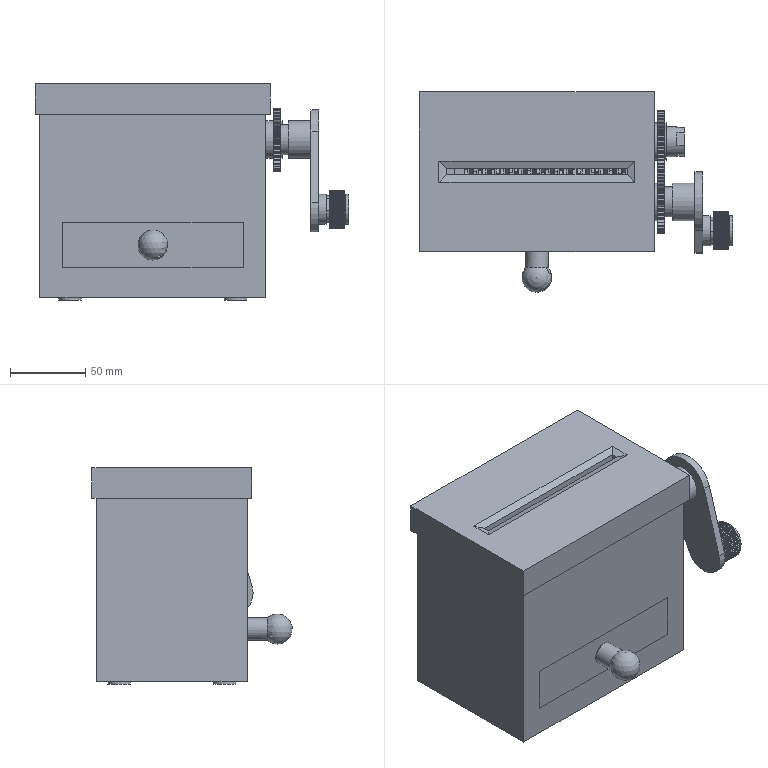Assembly | NX | mm | 9 component files | 11 solids | 2096 faces | box 208 x 133 x 143.5 mm | volume 1028833 mm3 | plane 897 | cylinder 878 | other 320 | sphere 1 | commonest cylinder face diameters 50 x288 1 x288 37.5 x80 42 x80 20 x56 25 x54 18 x8 15 x6
Bill of materials:
unnamed part 1 | 2 |  | Cylindrical shaft with a row of about 18 thin, evenly spaced discs along most of its length. Each disc has notched/serrated edges. Plain shaft stubs extend from both ends; one stub is longer and stepped, with a circumferential line or groove near its end.
unnamed part 2 | 1 |  | Flat, tapered lever arm with rounded ends. A plain cylindrical boss sits on one face at the wider end. A stepped cylindrical boss sits on the opposite face at the narrower end; it has a fine knurled or splined band and a smaller plain end cap.
unnamed part 3 | 1 |  | Open-top rectangular tray with thin walls and a flat floor. A short cylindrical stub ending in a sphere sticks out horizontally from the middle of one long outer wall. Small notches or tabs appear on the top edge of that wall, above the stub.
unnamed part 4 | 1 |  | Flat rectangular plate with one long, narrow through-slot running parallel to its long edge. The slot edges are chamfered or tapered on the top face.
unnamed part 5 | 2 |  | Spur gear with about 40 straight teeth around a large central bore. The bore has a small rectangular keyway notch. A cylindrical hub projects from one face.
unnamed part 6 | 1 |  | Thin, flat C-shaped ring of uniform thickness. Its two open ends finish in rounded lugs, and each lug has a small round hole.
unnamed part 7 | 1 |  | Open-top rectangular box with thin walls. Two U-shaped slots, open at the top edge, are cut into one short wall, with similar slots on the opposite short wall. A long rectangular window is cut near the bottom of one long wall. Small rectangular ledges or blocks sit at the top inner corners.
Mates:
1. fix | she_ji-1 1 component
2. touch align | she_ji-2 1 face | she_ji-1 1 face
3. touch align | she_ji-2 1 face | she_ji-1 1 face
4. touch align | she_ji-2 1 face | she_ji-1 1 face
5. touch align | she_ji-3 1 face | she_ji-1 1 face
6. touch align | she_ji-3 1 face | she_ji-1 1 face
7. touch align | she_ji-3 1 face | she_ji-1 1 face
8. touch align | she_ji-4 2 face | she_ji-1 1 face
9. touch align | she_ji-4 2 face | she_ji-1 1 face
10. touch align | she_ji-5 2 face | she_ji-4 2 face
11. touch align | she_ji-4 1 face | she_ji-1 1 face
12. distance | she_ji-4 2 face | she_ji-4 1 face
13. touch align | she_ji-5 2 face | she_ji-1 1 face
14. touch align | she_ji-4 2 face | she_ji-5 2 face
15. touch align | she_ji-5 1 face | she_ji-4 1 face
16. touch align | she_ji-5 1 face | she_ji-1 1 face
17. touch align | she_ji-5 1 face | she_ji-4 1 face
18. touch align | she_ji-5 1 face | she_ji-5 2 face
19. touch align | she_ji-6 1 face | she_ji-4 1 face
20. touch align | she_ji-6 1 face | she_ji-5 1 face
21. touch align | she_ji-7 1 face | she_ji-4 2 face
22. touch align | she_ji-7 1 face | she_ji-4 2 face
23. touch align | she_ji-7 1 face | she_ji-4 2 face